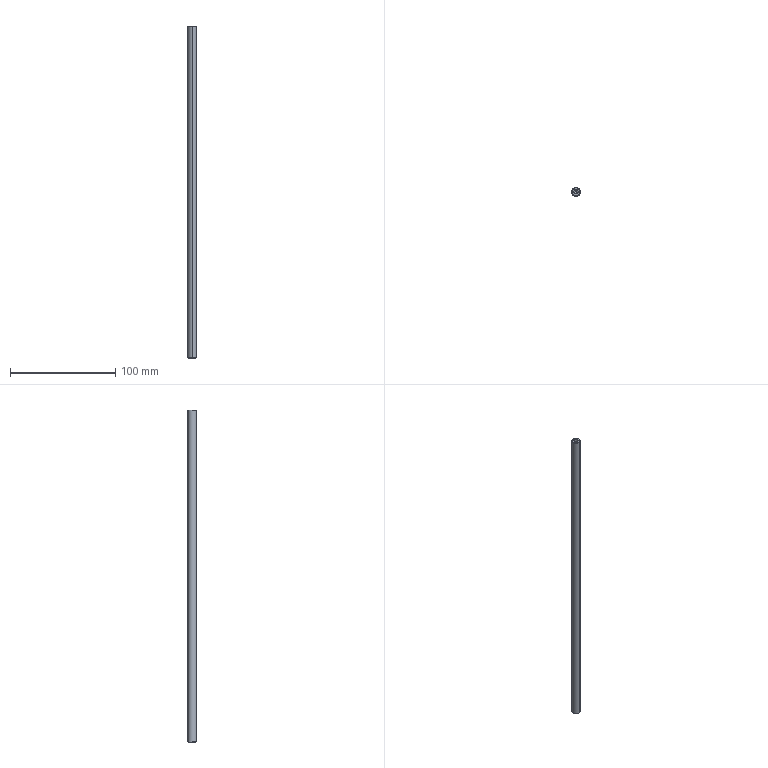Component | SolidWorks | LD101-02--Q1004-Q1-2-2 | 1 solid | 16 faces | box 8 x 8 x 315 mm | volume 15474 mm3 | cone 8 | cylinder 6 | plane 2 | commonest cylinder face diameters 4.2 x4 8 x2 | material 45
build123d program:
from build123d import *

# Parameters (mm, degrees)
SKETCH1_R           = 4
BOSS_EXTRUDE1_DEPTH = 157.5
CHAMFER1_SIZE       = 0.4


with BuildPart() as part:
    # Sketch1 → Boss-Extrude1 (new, symmetric)
    with BuildSketch(Plane.XY):
        Circle(SKETCH1_R)
    extrude(amount=BOSS_EXTRUDE1_DEPTH, both=True)

    # Sketch2 → M5 Tapped Hole1 (revolve, cut)
    with BuildSketch(Plane(origin=(0, 0, 157.5), x_dir=(0, -1, 0), z_dir=(1, 0, 0))):
        Polygon((0, 0), (0, 13.662), (2.1, 12.4), (2.1, 0), align=None)
    m5_tapped_hole1 = revolve(axis=Axis((0, 0, 163.85), (0, 0, -1)), mode=Mode.SUBTRACT)

    # Mirror1: M5 Tapped Hole1 across plane
    add(m5_tapped_hole1.mirror(Plane.XY), mode=Mode.SUBTRACT)

    # Chamfer1
    chamfer1_edges = [part.edges().sort_by_distance(p)[0] for p in [
        (-4, 0, -157.5),
        (-4, 0, 157.5),
    ]]
    chamfer(chamfer1_edges, length=CHAMFER1_SIZE)


solid = part.part

# Placed as in the assembly
solid = solid.moved(Location((79.71, -135.897, 146.257), (0, 0, 0)))
STEP:
#1=COLOUR_RGB('',0.7922,0.8196,0.9333);
#2=FILL_AREA_STYLE_COLOUR('',#1);
#3=FILL_AREA_STYLE('',(#2));
#4=SURFACE_STYLE_FILL_AREA(#3);
#5=SURFACE_SIDE_STYLE('',(#4));
#6=SURFACE_STYLE_USAGE(.BOTH.,#5);
#7=PRESENTATION_STYLE_ASSIGNMENT((#6));
#8=CARTESIAN_POINT('',(3.158,-5.491,-0.4427));
#9=VERTEX_POINT('',#8);
#10=CARTESIAN_POINT('',(3.118,-5.21,-0.4427));
#11=VERTEX_POINT('',#10);
#12=CARTESIAN_POINT('',(3.138,-5.35,-0.4427));
#13=DIRECTION('',(0.,0.,-1.));
#14=DIRECTION('',(0.1432,-0.9897,0.));
#15=AXIS2_PLACEMENT_3D('',#12,#13,#14);
#16=CIRCLE('',#15,0.1417);
#17=EDGE_CURVE('',#9,#11,#16,.T.);
#18=ORIENTED_EDGE('',*,*,#17,.F.);
#19=CARTESIAN_POINT('',(3.161,-5.506,-0.4269));
#20=VERTEX_POINT('',#19);
#21=CARTESIAN_POINT('',(3.158,-5.491,-0.4427));
#22=DIRECTION('',(0.1012,-0.6998,0.7071));
#23=VECTOR('',#22,39.37);
#24=LINE('',#21,#23);
#25=EDGE_CURVE('',#9,#20,#24,.T.);
#26=ORIENTED_EDGE('',*,*,#25,.T.);
#27=CARTESIAN_POINT('',(3.116,-5.194,-0.4269));
#28=VERTEX_POINT('',#27);
#29=CARTESIAN_POINT('',(3.138,-5.35,-0.4269));
#30=DIRECTION('',(-0.,-0.,1.));
#31=DIRECTION('',(0.1432,-0.9897,0.));
#32=AXIS2_PLACEMENT_3D('',#29,#30,#31);
#33=CIRCLE('',#32,0.1575);
#34=EDGE_CURVE('',#28,#20,#33,.T.);
#35=ORIENTED_EDGE('',*,*,#34,.F.);
#36=CARTESIAN_POINT('',(3.118,-5.21,-0.4427));
#37=DIRECTION('',(-0.1012,0.6998,0.7071));
#38=VECTOR('',#37,39.37);
#39=LINE('',#36,#38);
#40=EDGE_CURVE('',#11,#28,#39,.T.);
#41=ORIENTED_EDGE('',*,*,#40,.F.);
#42=EDGE_LOOP('',(#18,#26,#35,#41));
#43=FACE_OUTER_BOUND('',#42,.T.);
#44=CARTESIAN_POINT('',(3.138,-5.35,-0.4427));
#45=DIRECTION('',(-0.,-0.,1.));
#46=DIRECTION('',(-0.1432,0.9897,0.));
#47=AXIS2_PLACEMENT_3D('',#44,#45,#46);
#48=CONICAL_SURFACE('',#47,0.1417,0.7854);
#49=ADVANCED_FACE('',(#43),#48,.T.);
#50=CARTESIAN_POINT('',(3.118,-5.21,11.959));
#51=VERTEX_POINT('',#50);
#52=CARTESIAN_POINT('',(3.158,-5.491,11.959));
#53=VERTEX_POINT('',#52);
#54=CARTESIAN_POINT('',(3.138,-5.35,11.959));
#55=DIRECTION('',(-0.,-0.,1.));
#56=DIRECTION('',(0.1432,-0.9897,0.));
#57=AXIS2_PLACEMENT_3D('',#54,#55,#56);
#58=CIRCLE('',#57,0.1417);
#59=EDGE_CURVE('',#51,#53,#58,.T.);
#60=ORIENTED_EDGE('',*,*,#59,.F.);
#61=CARTESIAN_POINT('',(3.116,-5.194,11.943));
#62=VERTEX_POINT('',#61);
#63=CARTESIAN_POINT('',(3.116,-5.194,11.943));
#64=DIRECTION('',(-0.1012,0.6998,-0.7071));
#65=VECTOR('',#64,39.37);
#66=LINE('',#63,#65);
#67=EDGE_CURVE('',#51,#62,#66,.T.);
#68=ORIENTED_EDGE('',*,*,#67,.T.);
#69=CARTESIAN_POINT('',(3.161,-5.506,11.943));
#70=VERTEX_POINT('',#69);
#71=CARTESIAN_POINT('',(3.138,-5.35,11.943));
#72=DIRECTION('',(0.,0.,-1.));
#73=DIRECTION('',(0.1432,-0.9897,0.));
#74=AXIS2_PLACEMENT_3D('',#71,#72,#73);
#75=CIRCLE('',#74,0.1575);
#76=EDGE_CURVE('',#70,#62,#75,.T.);
#77=ORIENTED_EDGE('',*,*,#76,.F.);
#78=CARTESIAN_POINT('',(3.161,-5.506,11.943));
#79=DIRECTION('',(0.1012,-0.6998,-0.7071));
#80=VECTOR('',#79,39.37);
#81=LINE('',#78,#80);
#82=EDGE_CURVE('',#53,#70,#81,.T.);
#83=ORIENTED_EDGE('',*,*,#82,.F.);
#84=EDGE_LOOP('',(#60,#68,#77,#83));
#85=FACE_OUTER_BOUND('',#84,.T.);
#86=CARTESIAN_POINT('',(3.138,-5.35,11.943));
#87=DIRECTION('',(0.,0.,-1.));
#88=DIRECTION('',(0.1432,-0.9897,0.));
#89=AXIS2_PLACEMENT_3D('',#86,#87,#88);
#90=CONICAL_SURFACE('',#89,0.1575,0.7854);
#91=ADVANCED_FACE('',(#85),#90,.T.);
#92=CARTESIAN_POINT('',(3.15,-5.432,11.471));
#93=VERTEX_POINT('',#92);
#94=CARTESIAN_POINT('',(3.126,-5.268,11.471));
#95=VERTEX_POINT('',#94);
#96=CARTESIAN_POINT('',(3.138,-5.35,11.471));
#97=DIRECTION('',(-0.,-0.,1.));
#98=DIRECTION('',(-0.1432,0.9897,0.));
#99=AXIS2_PLACEMENT_3D('',#96,#97,#98);
#100=CIRCLE('',#99,0.08268);
#101=EDGE_CURVE('',#93,#95,#100,.T.);
#102=ORIENTED_EDGE('',*,*,#101,.F.);
#103=CARTESIAN_POINT('',(3.15,-5.432,11.959));
#104=VERTEX_POINT('',#103);
#105=CARTESIAN_POINT('',(3.15,-5.432,11.959));
#106=DIRECTION('',(-0.,-0.,1.));
#107=VECTOR('',#106,39.37);
#108=LINE('',#105,#107);
#109=EDGE_CURVE('',#93,#104,#108,.T.);
#110=ORIENTED_EDGE('',*,*,#109,.T.);
#111=CARTESIAN_POINT('',(3.126,-5.268,11.959));
#112=VERTEX_POINT('',#111);
#113=CARTESIAN_POINT('',(3.138,-5.35,11.959));
#114=DIRECTION('',(-0.,-0.,1.));
#115=DIRECTION('',(-0.1432,0.9897,0.));
#116=AXIS2_PLACEMENT_3D('',#113,#114,#115);
#117=CIRCLE('',#116,0.08268);
#118=EDGE_CURVE('',#104,#112,#117,.T.);
#119=ORIENTED_EDGE('',*,*,#118,.T.);
#120=CARTESIAN_POINT('',(3.126,-5.268,11.959));
#121=DIRECTION('',(-0.,-0.,1.));
#122=VECTOR('',#121,39.37);
#123=LINE('',#120,#122);
#124=EDGE_CURVE('',#95,#112,#123,.T.);
#125=ORIENTED_EDGE('',*,*,#124,.F.);
#126=EDGE_LOOP('',(#102,#110,#119,#125));
#127=FACE_OUTER_BOUND('',#126,.T.);
#128=CARTESIAN_POINT('',(3.138,-5.35,11.959));
#129=DIRECTION('',(-0.,-0.,1.));
#130=DIRECTION('',(-0.1432,0.9897,0.));
#131=AXIS2_PLACEMENT_3D('',#128,#129,#130);
#132=CYLINDRICAL_SURFACE('',#131,0.08268);
#133=ADVANCED_FACE('',(#127),#132,.F.);
#134=CARTESIAN_POINT('',(3.138,-5.35,11.421));
#135=VERTEX_POINT('',#134);
#136=CARTESIAN_POINT('',(3.126,-5.268,11.471));
#137=DIRECTION('',(-0.1227,0.8483,0.515));
#138=VECTOR('',#137,39.37);
#139=LINE('',#136,#138);
#140=EDGE_CURVE('',#135,#95,#139,.T.);
#141=ORIENTED_EDGE('',*,*,#140,.F.);
#142=CARTESIAN_POINT('',(3.15,-5.432,11.471));
#143=DIRECTION('',(0.1227,-0.8483,0.515));
#144=VECTOR('',#143,39.37);
#145=LINE('',#142,#144);
#146=EDGE_CURVE('',#135,#93,#145,.T.);
#147=ORIENTED_EDGE('',*,*,#146,.T.);
#148=ORIENTED_EDGE('',*,*,#101,.T.);
#149=EDGE_LOOP('',(#141,#147,#148));
#150=FACE_OUTER_BOUND('',#149,.T.);
#151=CARTESIAN_POINT('',(3.138,-5.35,11.471));
#152=DIRECTION('',(-0.,-0.,1.));
#153=DIRECTION('',(-0.1432,0.9897,0.));
#154=AXIS2_PLACEMENT_3D('',#151,#152,#153);
#155=CONICAL_SURFACE('',#154,0.08268,1.03);
#156=ADVANCED_FACE('',(#150),#155,.F.);
#157=CARTESIAN_POINT('',(3.126,-5.268,0.04554));
#158=VERTEX_POINT('',#157);
#159=CARTESIAN_POINT('',(3.15,-5.432,0.04554));
#160=VERTEX_POINT('',#159);
#161=CARTESIAN_POINT('',(3.138,-5.35,0.04554));
#162=DIRECTION('',(0.,0.,-1.));
#163=DIRECTION('',(0.1432,-0.9897,0.));
#164=AXIS2_PLACEMENT_3D('',#161,#162,#163);
#165=CIRCLE('',#164,0.08268);
#166=EDGE_CURVE('',#158,#160,#165,.T.);
#167=ORIENTED_EDGE('',*,*,#166,.F.);
#168=CARTESIAN_POINT('',(3.126,-5.268,-0.4427));
#169=VERTEX_POINT('',#168);
#170=CARTESIAN_POINT('',(3.126,-5.268,-0.4427));
#171=DIRECTION('',(0.,0.,-1.));
#172=VECTOR('',#171,39.37);
#173=LINE('',#170,#172);
#174=EDGE_CURVE('',#158,#169,#173,.T.);
#175=ORIENTED_EDGE('',*,*,#174,.T.);
#176=CARTESIAN_POINT('',(3.15,-5.432,-0.4427));
#177=VERTEX_POINT('',#176);
#178=CARTESIAN_POINT('',(3.138,-5.35,-0.4427));
#179=DIRECTION('',(0.,0.,-1.));
#180=DIRECTION('',(0.1432,-0.9897,0.));
#181=AXIS2_PLACEMENT_3D('',#178,#179,#180);
#182=CIRCLE('',#181,0.08268);
#183=EDGE_CURVE('',#169,#177,#182,.T.);
#184=ORIENTED_EDGE('',*,*,#183,.T.);
#185=CARTESIAN_POINT('',(3.15,-5.432,-0.4427));
#186=DIRECTION('',(0.,0.,-1.));
#187=VECTOR('',#186,39.37);
#188=LINE('',#185,#187);
#189=EDGE_CURVE('',#160,#177,#188,.T.);
#190=ORIENTED_EDGE('',*,*,#189,.F.);
#191=EDGE_LOOP('',(#167,#175,#184,#190));
#192=FACE_OUTER_BOUND('',#191,.T.);
#193=CARTESIAN_POINT('',(3.138,-5.35,-0.4427));
#194=DIRECTION('',(0.,0.,-1.));
#195=DIRECTION('',(0.1432,-0.9897,0.));
#196=AXIS2_PLACEMENT_3D('',#193,#194,#195);
#197=CYLINDRICAL_SURFACE('',#196,0.08268);
#198=ADVANCED_FACE('',(#192),#197,.F.);
#199=CARTESIAN_POINT('',(3.138,-5.35,0.09521));
#200=VERTEX_POINT('',#199);
#201=CARTESIAN_POINT('',(3.15,-5.432,0.04554));
#202=DIRECTION('',(0.1227,-0.8483,-0.515));
#203=VECTOR('',#202,39.37);
#204=LINE('',#201,#203);
#205=EDGE_CURVE('',#200,#160,#204,.T.);
#206=ORIENTED_EDGE('',*,*,#205,.F.);
#207=CARTESIAN_POINT('',(3.126,-5.268,0.04554));
#208=DIRECTION('',(-0.1227,0.8483,-0.515));
#209=VECTOR('',#208,39.37);
#210=LINE('',#207,#209);
#211=EDGE_CURVE('',#200,#158,#210,.T.);
#212=ORIENTED_EDGE('',*,*,#211,.T.);
#213=ORIENTED_EDGE('',*,*,#166,.T.);
#214=EDGE_LOOP('',(#206,#212,#213));
#215=FACE_OUTER_BOUND('',#214,.T.);
#216=CARTESIAN_POINT('',(3.138,-5.35,0.04554));
#217=DIRECTION('',(0.,0.,-1.));
#218=DIRECTION('',(0.1432,-0.9897,0.));
#219=AXIS2_PLACEMENT_3D('',#216,#217,#218);
#220=CONICAL_SURFACE('',#219,0.08268,1.03);
#221=ADVANCED_FACE('',(#215),#220,.F.);
#222=ORIENTED_EDGE('',*,*,#34,.T.);
#223=CARTESIAN_POINT('',(3.161,-5.506,-0.4427));
#224=DIRECTION('',(-0.,-0.,1.));
#225=VECTOR('',#224,39.37);
#226=LINE('',#223,#225);
#227=EDGE_CURVE('',#20,#70,#226,.T.);
#228=ORIENTED_EDGE('',*,*,#227,.T.);
#229=ORIENTED_EDGE('',*,*,#76,.T.);
#230=CARTESIAN_POINT('',(3.116,-5.194,-0.4427));
#231=DIRECTION('',(-0.,-0.,1.));
#232=VECTOR('',#231,39.37);
#233=LINE('',#230,#232);
#234=EDGE_CURVE('',#28,#62,#233,.T.);
#235=ORIENTED_EDGE('',*,*,#234,.F.);
#236=EDGE_LOOP('',(#222,#228,#229,#235));
#237=FACE_OUTER_BOUND('',#236,.T.);
#238=CARTESIAN_POINT('',(3.138,-5.35,-0.4427));
#239=DIRECTION('',(-0.,-0.,1.));
#240=DIRECTION('',(-0.1432,0.9897,0.));
#241=AXIS2_PLACEMENT_3D('',#238,#239,#240);
#242=CYLINDRICAL_SURFACE('',#241,0.1575);
#243=ADVANCED_FACE('',(#237),#242,.T.);
#244=ORIENTED_EDGE('',*,*,#227,.F.);
#245=CARTESIAN_POINT('',(3.138,-5.35,-0.4269));
#246=DIRECTION('',(-0.,-0.,1.));
#247=DIRECTION('',(0.1432,-0.9897,0.));
#248=AXIS2_PLACEMENT_3D('',#245,#246,#247);
#249=CIRCLE('',#248,0.1575);
#250=EDGE_CURVE('',#20,#28,#249,.T.);
#251=ORIENTED_EDGE('',*,*,#250,.T.);
#252=ORIENTED_EDGE('',*,*,#234,.T.);
#253=CARTESIAN_POINT('',(3.138,-5.35,11.943));
#254=DIRECTION('',(0.,0.,-1.));
#255=DIRECTION('',(0.1432,-0.9897,0.));
#256=AXIS2_PLACEMENT_3D('',#253,#254,#255);
#257=CIRCLE('',#256,0.1575);
#258=EDGE_CURVE('',#62,#70,#257,.T.);
#259=ORIENTED_EDGE('',*,*,#258,.T.);
#260=EDGE_LOOP('',(#244,#251,#252,#259));
#261=FACE_OUTER_BOUND('',#260,.T.);
#262=CARTESIAN_POINT('',(3.138,-5.35,-0.4427));
#263=DIRECTION('',(-0.,-0.,1.));
#264=DIRECTION('',(-0.1432,0.9897,0.));
#265=AXIS2_PLACEMENT_3D('',#262,#263,#264);
#266=CYLINDRICAL_SURFACE('',#265,0.1575);
#267=ADVANCED_FACE('',(#261),#266,.T.);
#268=CARTESIAN_POINT('',(3.138,-5.35,-0.4427));
#269=DIRECTION('',(0.,0.,-1.));
#270=DIRECTION('',(0.1432,-0.9897,0.));
#271=AXIS2_PLACEMENT_3D('',#268,#269,#270);
#272=CIRCLE('',#271,0.1417);
#273=EDGE_CURVE('',#11,#9,#272,.T.);
#274=ORIENTED_EDGE('',*,*,#273,.T.);
#275=ORIENTED_EDGE('',*,*,#17,.T.);
#276=EDGE_LOOP('',(#274,#275));
#277=FACE_OUTER_BOUND('',#276,.T.);
#278=CARTESIAN_POINT('',(3.138,-5.35,-0.4427));
#279=DIRECTION('',(0.,0.,-1.));
#280=DIRECTION('',(0.1432,-0.9897,0.));
#281=AXIS2_PLACEMENT_3D('',#278,#279,#280);
#282=CIRCLE('',#281,0.08268);
#283=EDGE_CURVE('',#177,#169,#282,.T.);
#284=ORIENTED_EDGE('',*,*,#283,.F.);
#285=ORIENTED_EDGE('',*,*,#183,.F.);
#286=EDGE_LOOP('',(#284,#285));
#287=FACE_BOUND('',#286,.T.);
#288=CARTESIAN_POINT('',(3.138,-5.35,-0.4427));
#289=DIRECTION('',(0.,0.,-1.));
#290=DIRECTION('',(0.1432,-0.9897,-0.));
#291=AXIS2_PLACEMENT_3D('',#288,#289,#290);
#292=PLANE('',#291);
#293=ADVANCED_FACE('',(#277,#287),#292,.T.);
#294=CARTESIAN_POINT('',(3.138,-5.35,11.959));
#295=DIRECTION('',(-0.,-0.,1.));
#296=DIRECTION('',(0.1432,-0.9897,0.));
#297=AXIS2_PLACEMENT_3D('',#294,#295,#296);
#298=CIRCLE('',#297,0.1417);
#299=EDGE_CURVE('',#53,#51,#298,.T.);
#300=ORIENTED_EDGE('',*,*,#299,.T.);
#301=ORIENTED_EDGE('',*,*,#59,.T.);
#302=EDGE_LOOP('',(#300,#301));
#303=FACE_OUTER_BOUND('',#302,.T.);
#304=CARTESIAN_POINT('',(3.138,-5.35,11.959));
#305=DIRECTION('',(-0.,-0.,1.));
#306=DIRECTION('',(-0.1432,0.9897,0.));
#307=AXIS2_PLACEMENT_3D('',#304,#305,#306);
#308=CIRCLE('',#307,0.08268);
#309=EDGE_CURVE('',#112,#104,#308,.T.);
#310=ORIENTED_EDGE('',*,*,#309,.F.);
#311=ORIENTED_EDGE('',*,*,#118,.F.);
#312=EDGE_LOOP('',(#310,#311));
#313=FACE_BOUND('',#312,.T.);
#314=CARTESIAN_POINT('',(3.138,-5.35,11.959));
#315=DIRECTION('',(0.,0.,-1.));
#316=DIRECTION('',(0.1432,-0.9897,-0.));
#317=AXIS2_PLACEMENT_3D('',#314,#315,#316);
#318=PLANE('',#317);
#319=ADVANCED_FACE('',(#303,#313),#318,.F.);
#320=ORIENTED_EDGE('',*,*,#211,.F.);
#321=ORIENTED_EDGE('',*,*,#205,.T.);
#322=CARTESIAN_POINT('',(3.138,-5.35,0.04554));
#323=DIRECTION('',(0.,0.,-1.));
#324=DIRECTION('',(0.1432,-0.9897,0.));
#325=AXIS2_PLACEMENT_3D('',#322,#323,#324);
#326=CIRCLE('',#325,0.08268);
#327=EDGE_CURVE('',#160,#158,#326,.T.);
#328=ORIENTED_EDGE('',*,*,#327,.T.);
#329=EDGE_LOOP('',(#320,#321,#328));
#330=FACE_OUTER_BOUND('',#329,.T.);
#331=CARTESIAN_POINT('',(3.138,-5.35,0.04554));
#332=DIRECTION('',(0.,0.,-1.));
#333=DIRECTION('',(0.1432,-0.9897,0.));
#334=AXIS2_PLACEMENT_3D('',#331,#332,#333);
#335=CONICAL_SURFACE('',#334,0.08268,1.03);
#336=ADVANCED_FACE('',(#330),#335,.F.);
#337=ORIENTED_EDGE('',*,*,#174,.F.);
#338=ORIENTED_EDGE('',*,*,#327,.F.);
#339=ORIENTED_EDGE('',*,*,#189,.T.);
#340=ORIENTED_EDGE('',*,*,#283,.T.);
#341=EDGE_LOOP('',(#337,#338,#339,#340));
#342=FACE_OUTER_BOUND('',#341,.T.);
#343=CARTESIAN_POINT('',(3.138,-5.35,-0.4427));
#344=DIRECTION('',(0.,0.,-1.));
#345=DIRECTION('',(0.1432,-0.9897,0.));
#346=AXIS2_PLACEMENT_3D('',#343,#344,#345);
#347=CYLINDRICAL_SURFACE('',#346,0.08268);
#348=ADVANCED_FACE('',(#342),#347,.F.);
#349=ORIENTED_EDGE('',*,*,#146,.F.);
#350=ORIENTED_EDGE('',*,*,#140,.T.);
#351=CARTESIAN_POINT('',(3.138,-5.35,11.471));
#352=DIRECTION('',(-0.,-0.,1.));
#353=DIRECTION('',(-0.1432,0.9897,0.));
#354=AXIS2_PLACEMENT_3D('',#351,#352,#353);
#355=CIRCLE('',#354,0.08268);
#356=EDGE_CURVE('',#95,#93,#355,.T.);
#357=ORIENTED_EDGE('',*,*,#356,.T.);
#358=EDGE_LOOP('',(#349,#350,#357));
#359=FACE_OUTER_BOUND('',#358,.T.);
#360=CARTESIAN_POINT('',(3.138,-5.35,11.471));
#361=DIRECTION('',(-0.,-0.,1.));
#362=DIRECTION('',(-0.1432,0.9897,0.));
#363=AXIS2_PLACEMENT_3D('',#360,#361,#362);
#364=CONICAL_SURFACE('',#363,0.08268,1.03);
#365=ADVANCED_FACE('',(#359),#364,.F.);
#366=ORIENTED_EDGE('',*,*,#109,.F.);
#367=ORIENTED_EDGE('',*,*,#356,.F.);
#368=ORIENTED_EDGE('',*,*,#124,.T.);
#369=ORIENTED_EDGE('',*,*,#309,.T.);
#370=EDGE_LOOP('',(#366,#367,#368,#369));
#371=FACE_OUTER_BOUND('',#370,.T.);
#372=CARTESIAN_POINT('',(3.138,-5.35,11.959));
#373=DIRECTION('',(-0.,-0.,1.));
#374=DIRECTION('',(-0.1432,0.9897,0.));
#375=AXIS2_PLACEMENT_3D('',#372,#373,#374);
#376=CYLINDRICAL_SURFACE('',#375,0.08268);
#377=ADVANCED_FACE('',(#371),#376,.F.);
#378=ORIENTED_EDGE('',*,*,#67,.F.);
#379=ORIENTED_EDGE('',*,*,#299,.F.);
#380=ORIENTED_EDGE('',*,*,#82,.T.);
#381=ORIENTED_EDGE('',*,*,#258,.F.);
#382=EDGE_LOOP('',(#378,#379,#380,#381));
#383=FACE_OUTER_BOUND('',#382,.T.);
#384=CARTESIAN_POINT('',(3.138,-5.35,11.943));
#385=DIRECTION('',(0.,0.,-1.));
#386=DIRECTION('',(0.1432,-0.9897,0.));
#387=AXIS2_PLACEMENT_3D('',#384,#385,#386);
#388=CONICAL_SURFACE('',#387,0.1575,0.7854);
#389=ADVANCED_FACE('',(#383),#388,.T.);
#390=ORIENTED_EDGE('',*,*,#25,.F.);
#391=ORIENTED_EDGE('',*,*,#273,.F.);
#392=ORIENTED_EDGE('',*,*,#40,.T.);
#393=ORIENTED_EDGE('',*,*,#250,.F.);
#394=EDGE_LOOP('',(#390,#391,#392,#393));
#395=FACE_OUTER_BOUND('',#394,.T.);
#396=CARTESIAN_POINT('',(3.138,-5.35,-0.4427));
#397=DIRECTION('',(-0.,-0.,1.));
#398=DIRECTION('',(-0.1432,0.9897,0.));
#399=AXIS2_PLACEMENT_3D('',#396,#397,#398);
#400=CONICAL_SURFACE('',#399,0.1417,0.7854);
#401=ADVANCED_FACE('',(#395),#400,.T.);
#402=CLOSED_SHELL('',(#49,#91,#133,#156,#198,#221,#243,#267,#293,#319,#336,#348,#365,#377,#389,#401));
#403=MANIFOLD_SOLID_BREP('',#402);
#404=STYLED_ITEM('',(#7),#403);
#405=(LENGTH_UNIT()NAMED_UNIT(*)SI_UNIT($,.METRE.));
#406=LENGTH_MEASURE_WITH_UNIT(LENGTH_MEASURE(0.0254),#405);
#407=DIMENSIONAL_EXPONENTS(1.,0.,0.,0.,0.,0.,0.);
#408=(CONVERSION_BASED_UNIT('',#406)LENGTH_UNIT()NAMED_UNIT(#407));
#409=UNCERTAINTY_MEASURE_WITH_UNIT(LENGTH_MEASURE(0.00001),#408,'','');
#410=(NAMED_UNIT(*)PLANE_ANGLE_UNIT()SI_UNIT($,.RADIAN.));
#411=(NAMED_UNIT(*)SI_UNIT($,.STERADIAN.)SOLID_ANGLE_UNIT());
#412=(GEOMETRIC_REPRESENTATION_CONTEXT(3)GLOBAL_UNCERTAINTY_ASSIGNED_CONTEXT((#409))GLOBAL_UNIT_ASSIGNED_CONTEXT((#408,#410,#411))REPRESENTATION_CONTEXT('',''));
#413=MECHANICAL_DESIGN_GEOMETRIC_PRESENTATION_REPRESENTATION('',(#404),#412);
#414=PRESENTATION_LAYER_ASSIGNMENT('','',(#404));
#415=CARTESIAN_POINT('',(0.,0.,0.));
#416=DIRECTION('',(0.,0.,1.));
#417=DIRECTION('',(1.,0.,0.));
#418=AXIS2_PLACEMENT_3D('',#415,#416,#417);
#419=(LENGTH_UNIT()NAMED_UNIT(*)SI_UNIT($,.METRE.));
#420=LENGTH_MEASURE_WITH_UNIT(LENGTH_MEASURE(0.0254),#419);
#421=DIMENSIONAL_EXPONENTS(1.,0.,0.,0.,0.,0.,0.);
#422=(CONVERSION_BASED_UNIT('',#420)LENGTH_UNIT()NAMED_UNIT(#421));
#423=UNCERTAINTY_MEASURE_WITH_UNIT(LENGTH_MEASURE(0.00001),#422,'','');
#424=(NAMED_UNIT(*)PLANE_ANGLE_UNIT()SI_UNIT($,.RADIAN.));
#425=(NAMED_UNIT(*)SI_UNIT($,.STERADIAN.)SOLID_ANGLE_UNIT());
#426=(GEOMETRIC_REPRESENTATION_CONTEXT(3)GLOBAL_UNCERTAINTY_ASSIGNED_CONTEXT((#423))GLOBAL_UNIT_ASSIGNED_CONTEXT((#422,#424,#425))REPRESENTATION_CONTEXT('',''));
#427=ADVANCED_BREP_SHAPE_REPRESENTATION('',(#403,#418),#426);